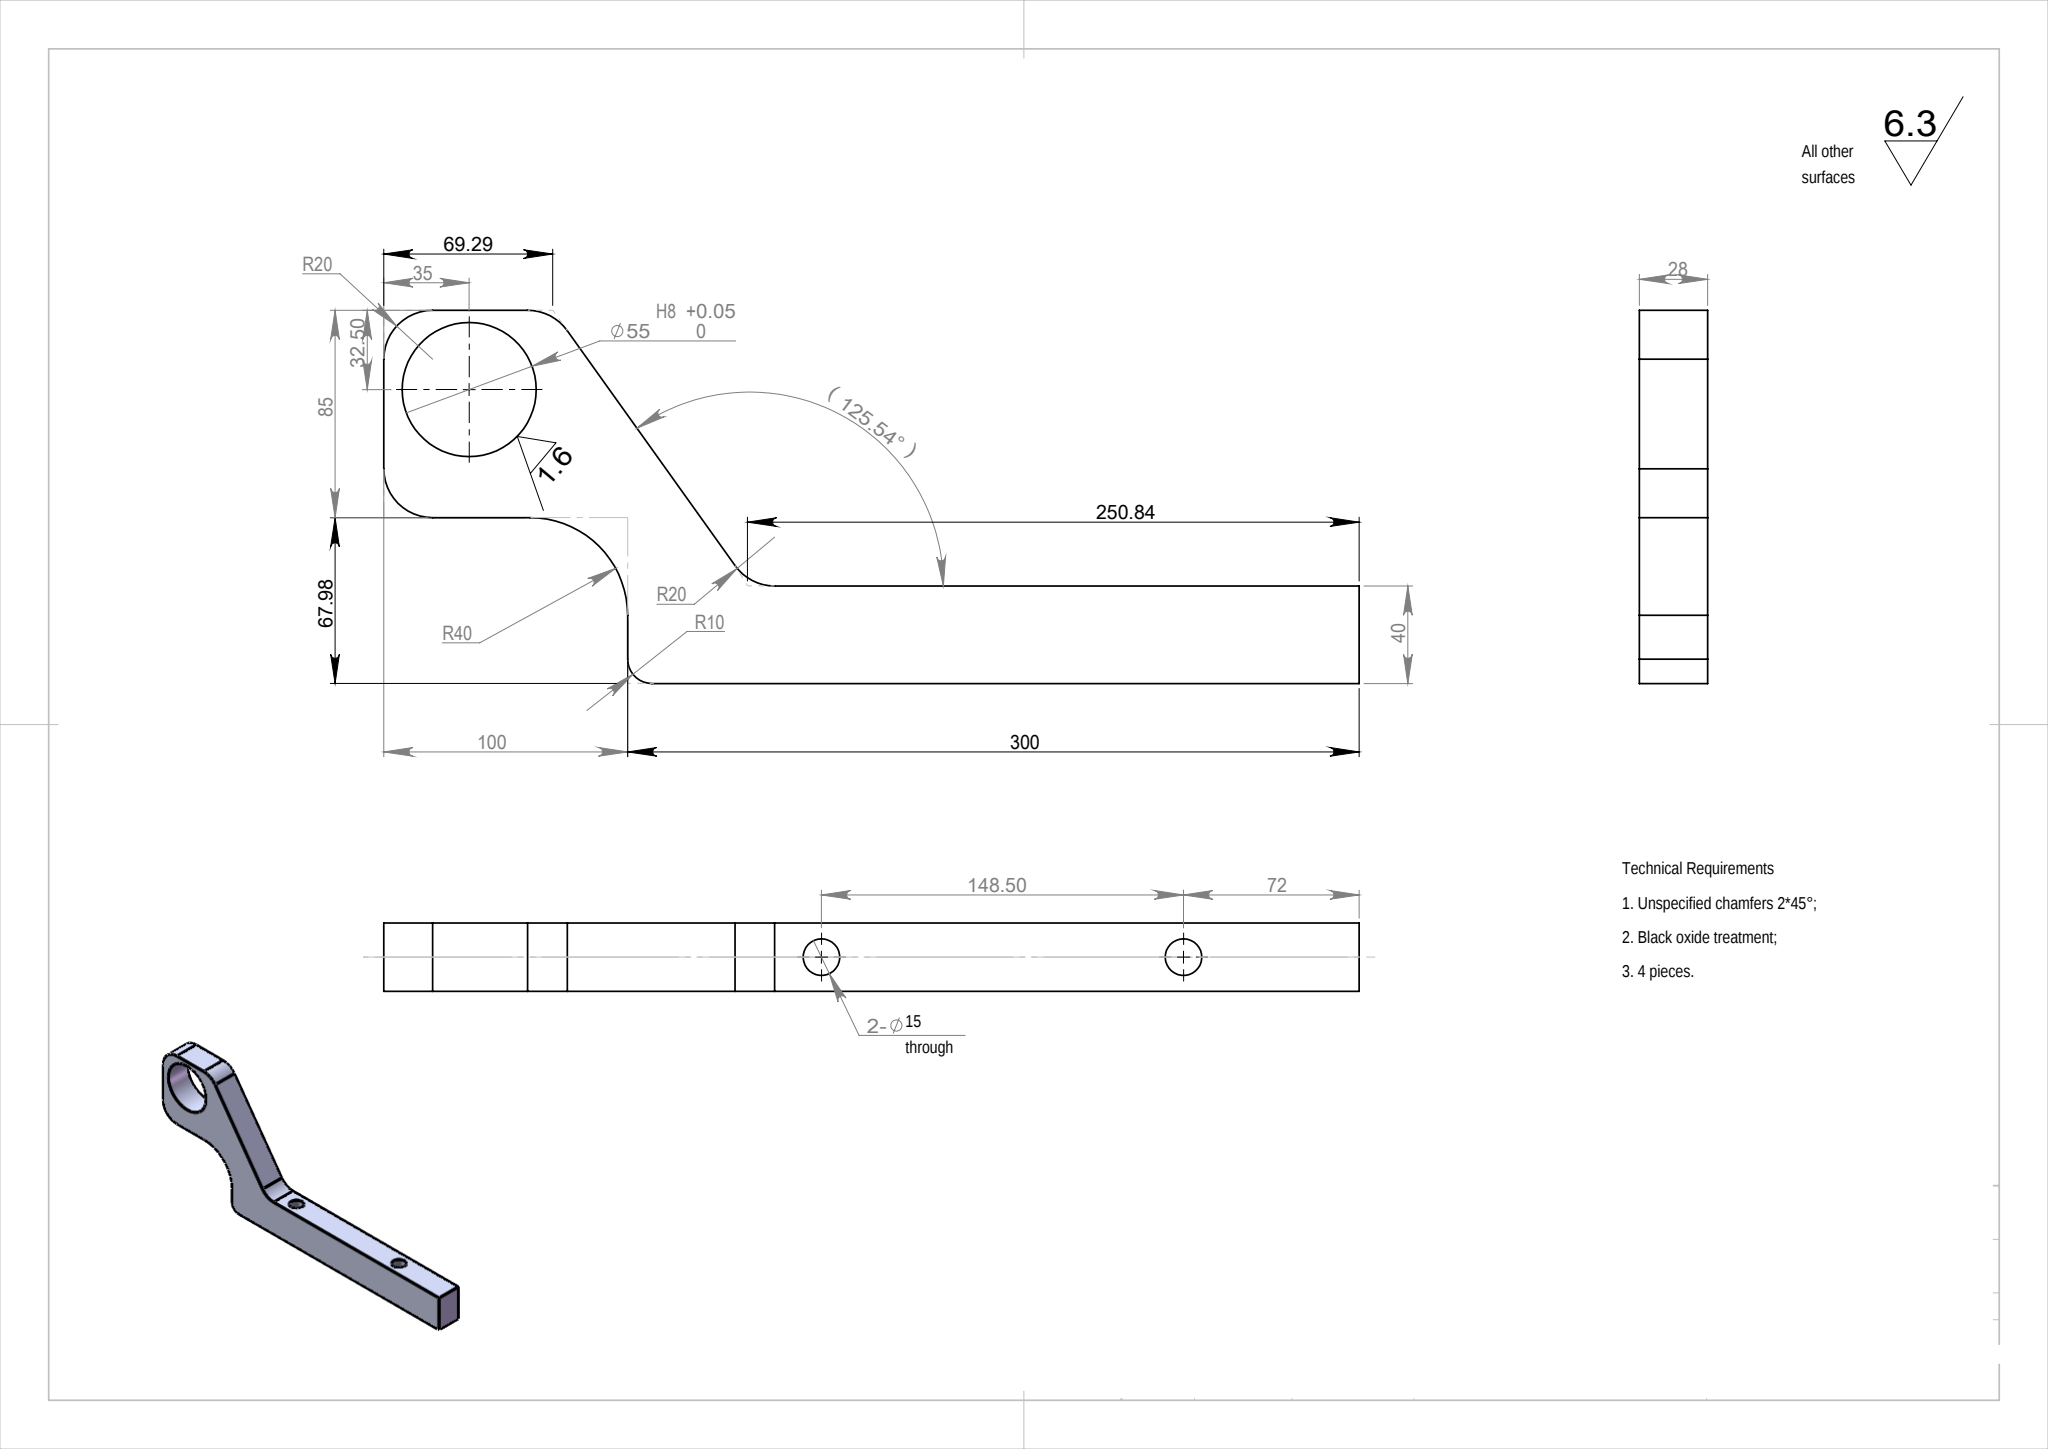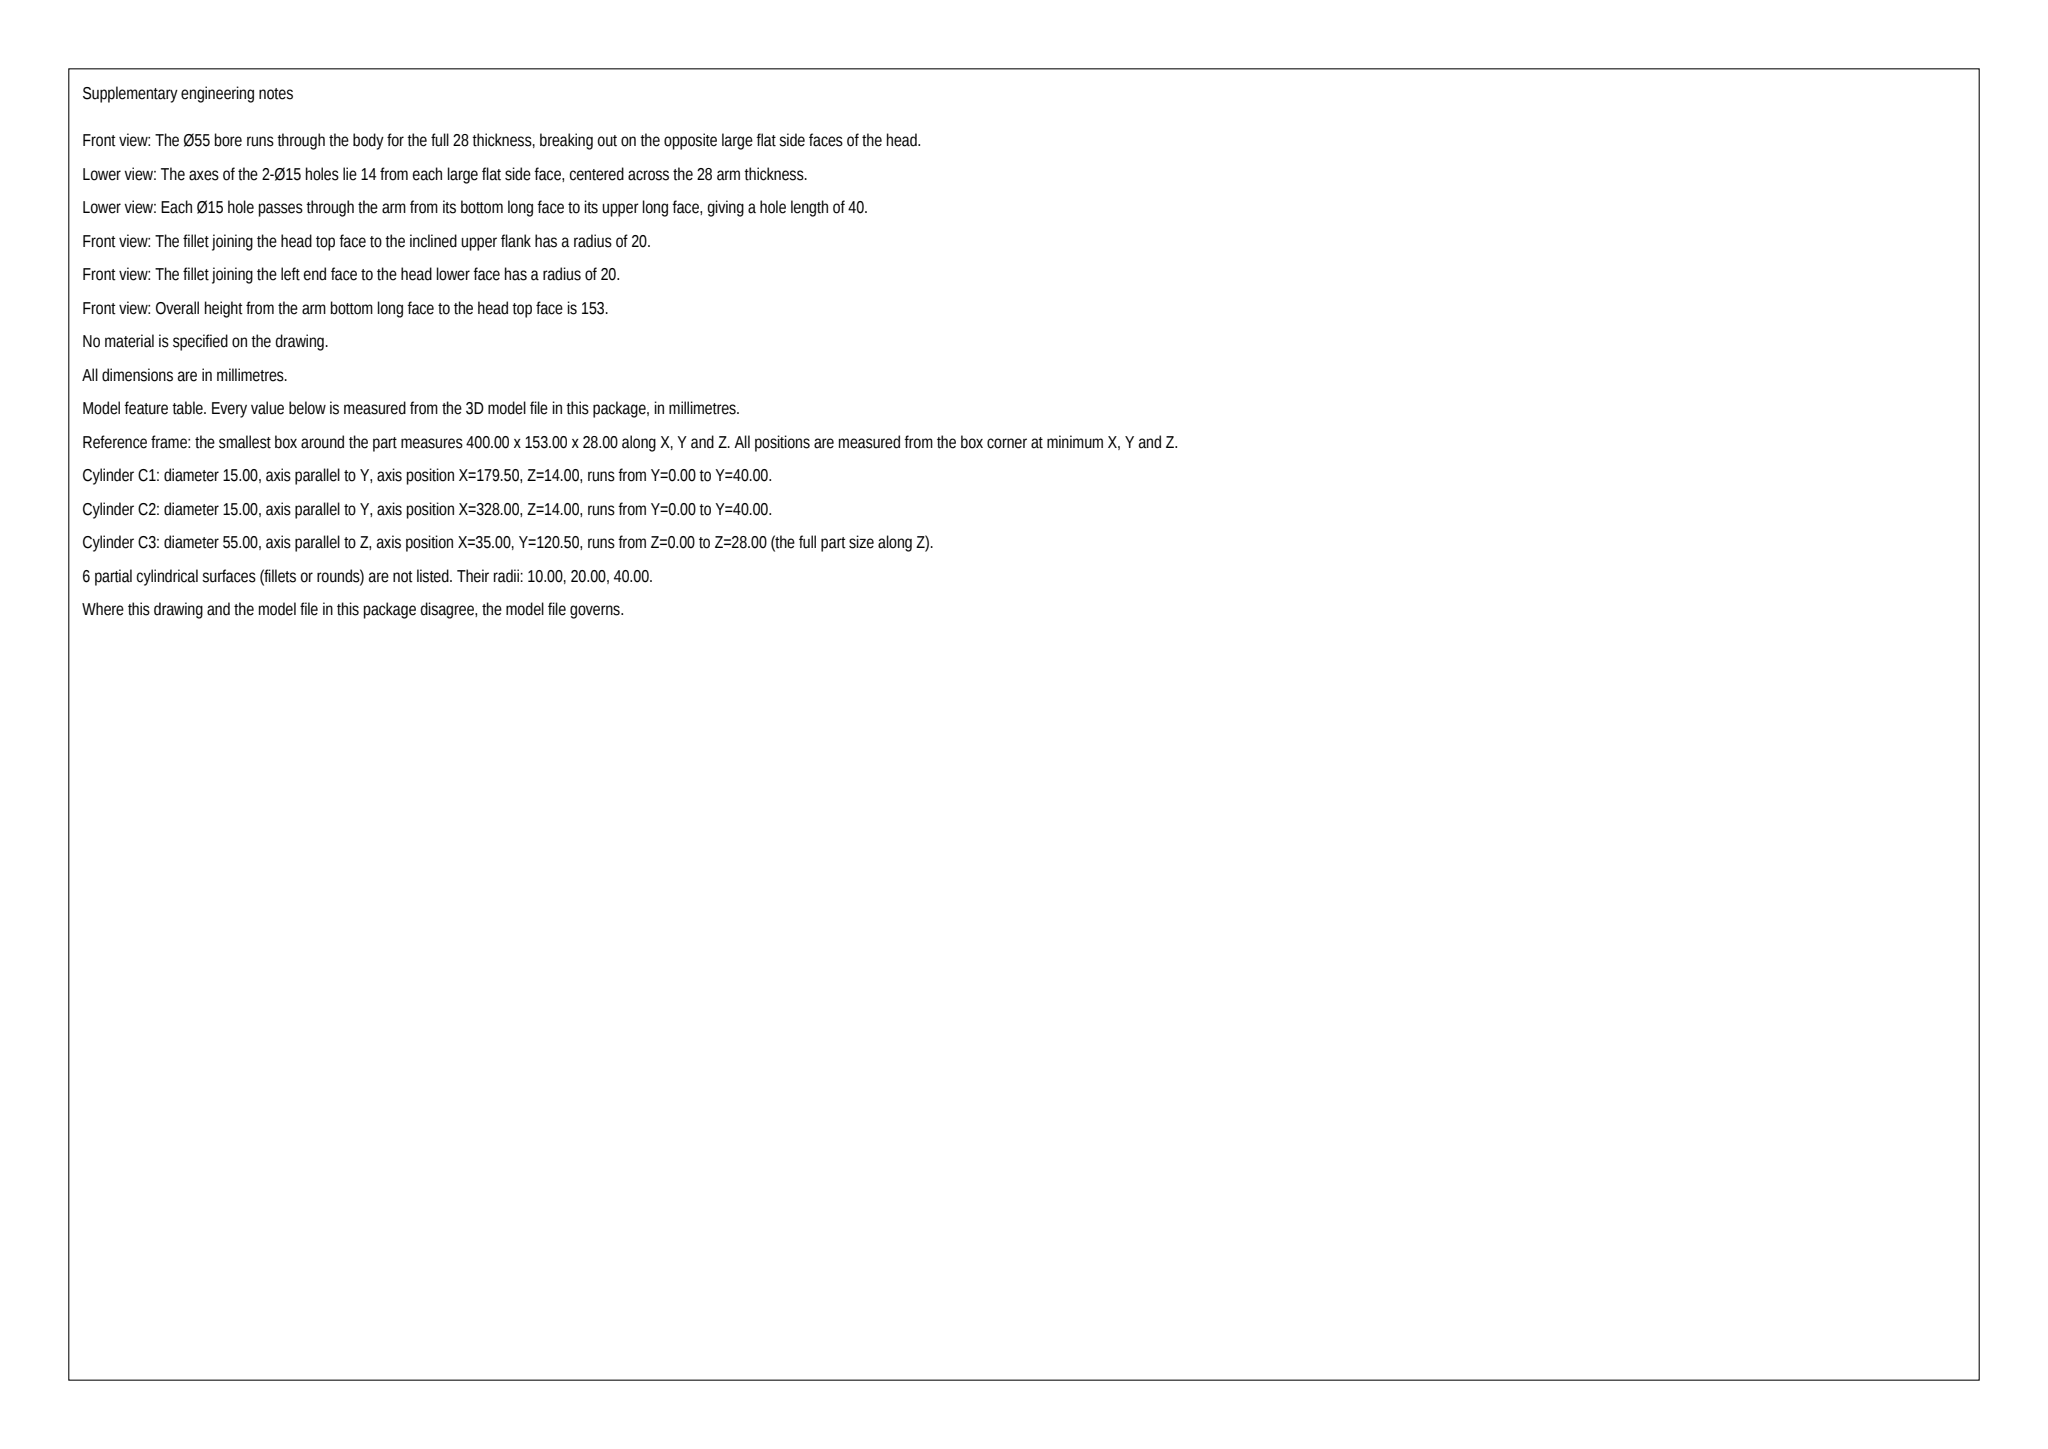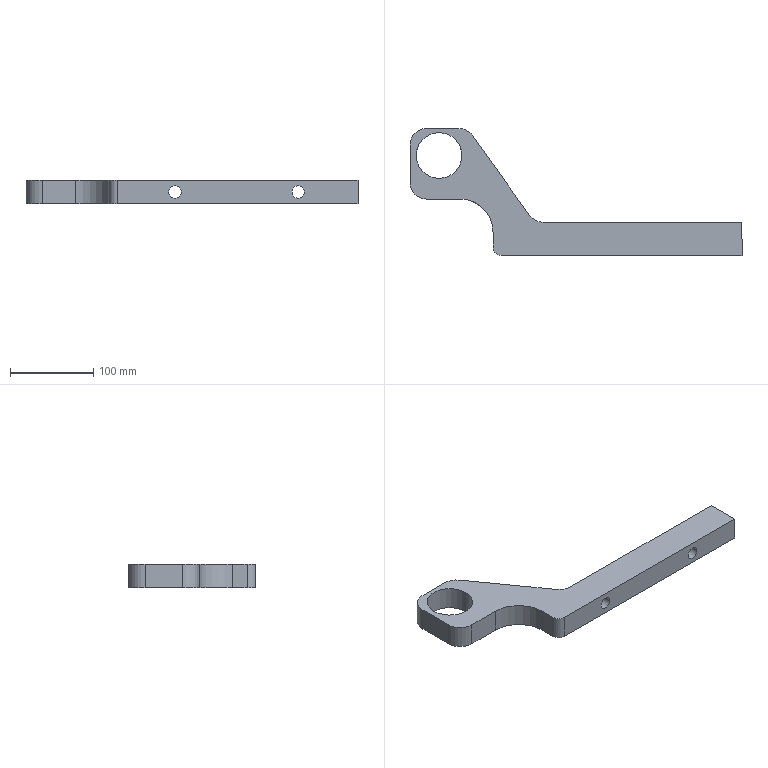Part | SolidWorks | mm | 1 solid | 22 faces | box 400 x 153 x 28 mm | volume 528056 mm3 | cylinder 12 | plane 10 | commonest cylinder face diameters 15 x4 40 x4 55 x2 80 x1 20 x1
Drawing notes:
FRONT VIEW: R20 AT LH END FACE/HEAD UNDERSIDE, CTR 20 FROM LH, 88 UP | from the solid: cylinder dia 40, axis z, pos (x=20, y=88), len 28 -> R20 tangent to planes x=0 and y=68
FRONT VIEW: R20 AT TOP EDGE/INCL EDGE, CTR 58.99 FROM LH, 133 UP | from the solid: cylinder dia 40, axis z, pos (x=58.99, y=133), len 28 -> R20 tangent to plane y=153 and inclined face
build123d program:
from build123d import *

# Parameters (mm, degrees)
BOSS_EXTRUDE1_DEPTH = 14
SKETCH2_R           = 5.5
CUT_EXTRUDE1_DEPTH  = 285.558
SKETCH3_R           = 27.5
CUT_EXTRUDE2_DEPTH  = 285.558
FILLET1_R           = 40
CUT_EXTRUDE5_DEPTH  = 285.558
FILLET3_R           = 20
FILLET5_R           = 10
CUT_EXTRUDE6_DEPTH  = 285.558
FILLET6_R           = 20
SKETCH13_R          = 7.5
CUT_EXTRUDE7_DEPTH  = 294.437


with BuildPart() as part:
    # Sketch1 → Boss-Extrude1 (new, symmetric)
    with BuildSketch(Plane.XY):
        Polygon((-150, 133), (0, 133), (0, 0), (250, 0), (250, -40), (-50, -40), (-50, 28), (-150, 28), align=None)
    extrude(amount=BOSS_EXTRUDE1_DEPTH, both=True)

    # Sketch2 → Cut-Extrude1 (cut, through all)
    with BuildSketch(Plane.XY.offset(14)):
        with Locations((-115, 80.5)):
            Circle(SKETCH2_R)
    extrude(amount=-CUT_EXTRUDE1_DEPTH, mode=Mode.SUBTRACT)

    # Sketch3 → Cut-Extrude2 (cut, through all)
    with BuildSketch(Plane(origin=(0, 0, 14), x_dir=(-1, 0, 0), z_dir=(0, 0, -1))):
        with Locations((115, 80.5)):
            Circle(SKETCH3_R)
    extrude(amount=CUT_EXTRUDE2_DEPTH, mode=Mode.SUBTRACT)

    # Fillet1
    fillet1_edges = [part.edges().sort_by_distance(p)[0] for p in [
        (-50, 28, 0),
    ]]
    fillet(fillet1_edges, radius=FILLET1_R)

    # Sketch10 → Cut-Extrude5 (cut, through all)
    with BuildSketch(Plane.XY.offset(14)):
        Polygon((-95, 133), (0, 0), (0, 133), align=None)
    extrude(amount=-CUT_EXTRUDE5_DEPTH, mode=Mode.SUBTRACT)

    # Fillet3
    fillet3_edges = [part.edges().sort_by_distance(p)[0] for p in [
        (0, 0, 0),
    ]]
    fillet(fillet3_edges, radius=FILLET3_R)

    # Fillet5
    fillet5_edges = [part.edges().sort_by_distance(p)[0] for p in [
        (-50, -40, 0),
    ]]
    fillet(fillet5_edges, radius=FILLET5_R)

    # Sketch11 → Cut-Extrude6 (cut, through all)
    with BuildSketch(Plane.XY.offset(14)):
        Polygon((-150, 113), (-80.714, 113), (-95, 133), (-150, 133), align=None)
    extrude(amount=-CUT_EXTRUDE6_DEPTH, mode=Mode.SUBTRACT)

    # Fillet6
    fillet6_edges = [part.edges().sort_by_distance(p)[0] for p in [
        (-150, 28, 0),
        (-150, 113, 0),
        (-80.714, 113, 0),
    ]]
    fillet(fillet6_edges, radius=FILLET6_R)

    # Sketch13 → Cut-Extrude7 (cut, through all)
    with BuildSketch(Plane.XZ.offset(40)):
        with Locations((29.5, 0)):
            Circle(SKETCH13_R)
        with Locations((178, 0)):
            Circle(SKETCH13_R)
    extrude(amount=-CUT_EXTRUDE7_DEPTH, mode=Mode.SUBTRACT)


solid = part.part
STEP:
#1=CARTESIAN_POINT('',(22.,0.,0.));
#2=VERTEX_POINT('',#1);
#3=CARTESIAN_POINT('',(37.,0.,0.));
#4=VERTEX_POINT('',#3);
#5=CARTESIAN_POINT('',(29.5,0.,0.));
#6=DIRECTION('',(0.,-1.,0.));
#7=DIRECTION('',(0.,0.,-1.));
#8=AXIS2_PLACEMENT_3D('',#5,#6,#7);
#9=CIRCLE('',#8,7.5);
#10=EDGE_CURVE('',#2,#4,#9,.T.);
#11=ORIENTED_EDGE('',*,*,#10,.F.);
#12=CARTESIAN_POINT('',(22.,-40.,0.));
#13=VERTEX_POINT('',#12);
#14=CARTESIAN_POINT('',(22.,113.,0.));
#15=DIRECTION('',(0.,-1.,0.));
#16=VECTOR('',#15,1000.);
#17=LINE('',#14,#16);
#18=EDGE_CURVE('',#2,#13,#17,.T.);
#19=ORIENTED_EDGE('',*,*,#18,.T.);
#20=CARTESIAN_POINT('',(37.,-40.,0.));
#21=VERTEX_POINT('',#20);
#22=CARTESIAN_POINT('',(29.5,-40.,0.));
#23=DIRECTION('',(0.,-1.,0.));
#24=DIRECTION('',(1.,0.,0.));
#25=AXIS2_PLACEMENT_3D('',#22,#23,#24);
#26=CIRCLE('',#25,7.5);
#27=EDGE_CURVE('',#13,#21,#26,.T.);
#28=ORIENTED_EDGE('',*,*,#27,.T.);
#29=CARTESIAN_POINT('',(37.,113.,0.));
#30=DIRECTION('',(0.,-1.,0.));
#31=VECTOR('',#30,1000.);
#32=LINE('',#29,#31);
#33=EDGE_CURVE('',#4,#21,#32,.T.);
#34=ORIENTED_EDGE('',*,*,#33,.F.);
#35=EDGE_LOOP('',(#11,#19,#28,#34));
#36=FACE_OUTER_BOUND('',#35,.T.);
#37=CARTESIAN_POINT('',(29.5,113.,0.));
#38=DIRECTION('',(0.,-1.,0.));
#39=DIRECTION('',(1.,0.,0.));
#40=AXIS2_PLACEMENT_3D('',#37,#38,#39);
#41=CYLINDRICAL_SURFACE('',#40,7.5);
#42=ADVANCED_FACE('',(#36),#41,.F.);
#43=CARTESIAN_POINT('',(170.5,0.,0.));
#44=VERTEX_POINT('',#43);
#45=CARTESIAN_POINT('',(185.5,0.,0.));
#46=VERTEX_POINT('',#45);
#47=CARTESIAN_POINT('',(178.,0.,0.));
#48=DIRECTION('',(0.,-1.,0.));
#49=DIRECTION('',(0.,0.,-1.));
#50=AXIS2_PLACEMENT_3D('',#47,#48,#49);
#51=CIRCLE('',#50,7.5);
#52=EDGE_CURVE('',#44,#46,#51,.T.);
#53=ORIENTED_EDGE('',*,*,#52,.F.);
#54=CARTESIAN_POINT('',(170.5,-40.,0.));
#55=VERTEX_POINT('',#54);
#56=CARTESIAN_POINT('',(170.5,113.,0.));
#57=DIRECTION('',(0.,-1.,0.));
#58=VECTOR('',#57,1000.);
#59=LINE('',#56,#58);
#60=EDGE_CURVE('',#44,#55,#59,.T.);
#61=ORIENTED_EDGE('',*,*,#60,.T.);
#62=CARTESIAN_POINT('',(185.5,-40.,0.));
#63=VERTEX_POINT('',#62);
#64=CARTESIAN_POINT('',(178.,-40.,0.));
#65=DIRECTION('',(0.,-1.,0.));
#66=DIRECTION('',(1.,0.,0.));
#67=AXIS2_PLACEMENT_3D('',#64,#65,#66);
#68=CIRCLE('',#67,7.5);
#69=EDGE_CURVE('',#55,#63,#68,.T.);
#70=ORIENTED_EDGE('',*,*,#69,.T.);
#71=CARTESIAN_POINT('',(185.5,113.,0.));
#72=DIRECTION('',(0.,-1.,0.));
#73=VECTOR('',#72,1000.);
#74=LINE('',#71,#73);
#75=EDGE_CURVE('',#46,#63,#74,.T.);
#76=ORIENTED_EDGE('',*,*,#75,.F.);
#77=EDGE_LOOP('',(#53,#61,#70,#76));
#78=FACE_OUTER_BOUND('',#77,.T.);
#79=CARTESIAN_POINT('',(178.,113.,0.));
#80=DIRECTION('',(0.,-1.,0.));
#81=DIRECTION('',(1.,0.,0.));
#82=AXIS2_PLACEMENT_3D('',#79,#80,#81);
#83=CYLINDRICAL_SURFACE('',#82,7.5);
#84=ADVANCED_FACE('',(#78),#83,.F.);
#85=CARTESIAN_POINT('',(-87.5,80.5,-14.));
#86=VERTEX_POINT('',#85);
#87=CARTESIAN_POINT('',(-142.5,80.5,-14.));
#88=VERTEX_POINT('',#87);
#89=CARTESIAN_POINT('',(-115.,80.5,-14.));
#90=DIRECTION('',(0.,0.,-1.));
#91=DIRECTION('',(-1.,0.,0.));
#92=AXIS2_PLACEMENT_3D('',#89,#90,#91);
#93=CIRCLE('',#92,27.5);
#94=EDGE_CURVE('',#86,#88,#93,.T.);
#95=ORIENTED_EDGE('',*,*,#94,.T.);
#96=CARTESIAN_POINT('',(-142.5,80.5,14.));
#97=VERTEX_POINT('',#96);
#98=CARTESIAN_POINT('',(-142.5,80.5,-14.));
#99=DIRECTION('',(0.,0.,1.));
#100=VECTOR('',#99,1000.);
#101=LINE('',#98,#100);
#102=EDGE_CURVE('',#88,#97,#101,.T.);
#103=ORIENTED_EDGE('',*,*,#102,.T.);
#104=CARTESIAN_POINT('',(-87.5,80.5,14.));
#105=VERTEX_POINT('',#104);
#106=CARTESIAN_POINT('',(-115.,80.5,14.));
#107=DIRECTION('',(0.,0.,-1.));
#108=DIRECTION('',(-1.,0.,0.));
#109=AXIS2_PLACEMENT_3D('',#106,#107,#108);
#110=CIRCLE('',#109,27.5);
#111=EDGE_CURVE('',#105,#97,#110,.T.);
#112=ORIENTED_EDGE('',*,*,#111,.F.);
#113=CARTESIAN_POINT('',(-87.5,80.5,-14.));
#114=DIRECTION('',(0.,0.,1.));
#115=VECTOR('',#114,1000.);
#116=LINE('',#113,#115);
#117=EDGE_CURVE('',#86,#105,#116,.T.);
#118=ORIENTED_EDGE('',*,*,#117,.F.);
#119=EDGE_LOOP('',(#95,#103,#112,#118));
#120=FACE_OUTER_BOUND('',#119,.T.);
#121=CARTESIAN_POINT('',(-115.,80.5,-14.));
#122=DIRECTION('',(0.,0.,1.));
#123=DIRECTION('',(1.,0.,0.));
#124=AXIS2_PLACEMENT_3D('',#121,#122,#123);
#125=CYLINDRICAL_SURFACE('',#124,27.5);
#126=ADVANCED_FACE('',(#120),#125,.F.);
#127=CARTESIAN_POINT('',(-150.,93.,14.));
#128=VERTEX_POINT('',#127);
#129=CARTESIAN_POINT('',(-150.,48.,14.));
#130=VERTEX_POINT('',#129);
#131=CARTESIAN_POINT('',(-150.,28.,14.));
#132=DIRECTION('',(-0.,-1.,0.));
#133=VECTOR('',#132,1000.);
#134=LINE('',#131,#133);
#135=EDGE_CURVE('',#128,#130,#134,.T.);
#136=ORIENTED_EDGE('',*,*,#135,.F.);
#137=CARTESIAN_POINT('',(-150.,93.,-14.));
#138=VERTEX_POINT('',#137);
#139=CARTESIAN_POINT('',(-150.,93.,14.));
#140=DIRECTION('',(0.,0.,-1.));
#141=VECTOR('',#140,1000.);
#142=LINE('',#139,#141);
#143=EDGE_CURVE('',#128,#138,#142,.T.);
#144=ORIENTED_EDGE('',*,*,#143,.T.);
#145=CARTESIAN_POINT('',(-150.,48.,-14.));
#146=VERTEX_POINT('',#145);
#147=CARTESIAN_POINT('',(-150.,28.,-14.));
#148=DIRECTION('',(-0.,-1.,0.));
#149=VECTOR('',#148,1000.);
#150=LINE('',#147,#149);
#151=EDGE_CURVE('',#138,#146,#150,.T.);
#152=ORIENTED_EDGE('',*,*,#151,.T.);
#153=CARTESIAN_POINT('',(-150.,48.,14.));
#154=DIRECTION('',(0.,0.,1.));
#155=VECTOR('',#154,1000.);
#156=LINE('',#153,#155);
#157=EDGE_CURVE('',#146,#130,#156,.T.);
#158=ORIENTED_EDGE('',*,*,#157,.T.);
#159=EDGE_LOOP('',(#136,#144,#152,#158));
#160=FACE_OUTER_BOUND('',#159,.T.);
#161=CARTESIAN_POINT('',(-150.,28.,14.));
#162=DIRECTION('',(1.,-0.,0.));
#163=DIRECTION('',(0.,1.,0.));
#164=AXIS2_PLACEMENT_3D('',#161,#162,#163);
#165=PLANE('',#164);
#166=ADVANCED_FACE('',(#160),#165,.F.);
#167=CARTESIAN_POINT('',(-130.,28.,14.));
#168=VERTEX_POINT('',#167);
#169=CARTESIAN_POINT('',(-90.,28.,14.));
#170=VERTEX_POINT('',#169);
#171=CARTESIAN_POINT('',(-50.,28.,14.));
#172=DIRECTION('',(1.,0.,0.));
#173=VECTOR('',#172,1000.);
#174=LINE('',#171,#173);
#175=EDGE_CURVE('',#168,#170,#174,.T.);
#176=ORIENTED_EDGE('',*,*,#175,.F.);
#177=CARTESIAN_POINT('',(-130.,28.,-14.));
#178=VERTEX_POINT('',#177);
#179=CARTESIAN_POINT('',(-130.,28.,14.));
#180=DIRECTION('',(0.,0.,-1.));
#181=VECTOR('',#180,1000.);
#182=LINE('',#179,#181);
#183=EDGE_CURVE('',#168,#178,#182,.T.);
#184=ORIENTED_EDGE('',*,*,#183,.T.);
#185=CARTESIAN_POINT('',(-90.,28.,-14.));
#186=VERTEX_POINT('',#185);
#187=CARTESIAN_POINT('',(-50.,28.,-14.));
#188=DIRECTION('',(1.,0.,0.));
#189=VECTOR('',#188,1000.);
#190=LINE('',#187,#189);
#191=EDGE_CURVE('',#178,#186,#190,.T.);
#192=ORIENTED_EDGE('',*,*,#191,.T.);
#193=CARTESIAN_POINT('',(-90.,28.,14.));
#194=DIRECTION('',(0.,0.,1.));
#195=VECTOR('',#194,1000.);
#196=LINE('',#193,#195);
#197=EDGE_CURVE('',#186,#170,#196,.T.);
#198=ORIENTED_EDGE('',*,*,#197,.T.);
#199=EDGE_LOOP('',(#176,#184,#192,#198));
#200=FACE_OUTER_BOUND('',#199,.T.);
#201=CARTESIAN_POINT('',(-50.,28.,14.));
#202=DIRECTION('',(-0.,1.,0.));
#203=DIRECTION('',(-1.,-0.,0.));
#204=AXIS2_PLACEMENT_3D('',#201,#202,#203);
#205=PLANE('',#204);
#206=ADVANCED_FACE('',(#200),#205,.F.);
#207=CARTESIAN_POINT('',(-50.,-12.,-14.));
#208=VERTEX_POINT('',#207);
#209=CARTESIAN_POINT('',(-50.,-30.,-14.));
#210=VERTEX_POINT('',#209);
#211=CARTESIAN_POINT('',(-50.,-40.,-14.));
#212=DIRECTION('',(0.,-1.,0.));
#213=VECTOR('',#212,1000.);
#214=LINE('',#211,#213);
#215=EDGE_CURVE('',#208,#210,#214,.T.);
#216=ORIENTED_EDGE('',*,*,#215,.T.);
#217=CARTESIAN_POINT('',(-50.,-30.,14.));
#218=VERTEX_POINT('',#217);
#219=CARTESIAN_POINT('',(-50.,-30.,14.));
#220=DIRECTION('',(0.,0.,1.));
#221=VECTOR('',#220,1000.);
#222=LINE('',#219,#221);
#223=EDGE_CURVE('',#210,#218,#222,.T.);
#224=ORIENTED_EDGE('',*,*,#223,.T.);
#225=CARTESIAN_POINT('',(-50.,-12.,14.));
#226=VERTEX_POINT('',#225);
#227=CARTESIAN_POINT('',(-50.,-40.,14.));
#228=DIRECTION('',(0.,-1.,0.));
#229=VECTOR('',#228,1000.);
#230=LINE('',#227,#229);
#231=EDGE_CURVE('',#226,#218,#230,.T.);
#232=ORIENTED_EDGE('',*,*,#231,.F.);
#233=CARTESIAN_POINT('',(-50.,-12.,-14.));
#234=DIRECTION('',(0.,0.,-1.));
#235=VECTOR('',#234,1000.);
#236=LINE('',#233,#235);
#237=EDGE_CURVE('',#226,#208,#236,.T.);
#238=ORIENTED_EDGE('',*,*,#237,.T.);
#239=EDGE_LOOP('',(#216,#224,#232,#238));
#240=FACE_OUTER_BOUND('',#239,.T.);
#241=CARTESIAN_POINT('',(-50.,-40.,14.));
#242=DIRECTION('',(1.,0.,0.));
#243=DIRECTION('',(-0.,1.,0.));
#244=AXIS2_PLACEMENT_3D('',#241,#242,#243);
#245=PLANE('',#244);
#246=ADVANCED_FACE('',(#240),#245,.F.);
#247=CARTESIAN_POINT('',(29.5,-40.,0.));
#248=DIRECTION('',(0.,-1.,0.));
#249=DIRECTION('',(1.,0.,0.));
#250=AXIS2_PLACEMENT_3D('',#247,#248,#249);
#251=CIRCLE('',#250,7.5);
#252=EDGE_CURVE('',#21,#13,#251,.T.);
#253=ORIENTED_EDGE('',*,*,#252,.F.);
#254=ORIENTED_EDGE('',*,*,#27,.F.);
#255=EDGE_LOOP('',(#253,#254));
#256=FACE_BOUND('',#255,.T.);
#257=CARTESIAN_POINT('',(178.,-40.,0.));
#258=DIRECTION('',(0.,-1.,0.));
#259=DIRECTION('',(1.,0.,0.));
#260=AXIS2_PLACEMENT_3D('',#257,#258,#259);
#261=CIRCLE('',#260,7.5);
#262=EDGE_CURVE('',#63,#55,#261,.T.);
#263=ORIENTED_EDGE('',*,*,#262,.F.);
#264=ORIENTED_EDGE('',*,*,#69,.F.);
#265=EDGE_LOOP('',(#263,#264));
#266=FACE_BOUND('',#265,.T.);
#267=CARTESIAN_POINT('',(-40.,-40.,14.));
#268=VERTEX_POINT('',#267);
#269=CARTESIAN_POINT('',(250.,-40.,14.));
#270=VERTEX_POINT('',#269);
#271=CARTESIAN_POINT('',(250.,-40.,14.));
#272=DIRECTION('',(1.,0.,0.));
#273=VECTOR('',#272,1000.);
#274=LINE('',#271,#273);
#275=EDGE_CURVE('',#268,#270,#274,.T.);
#276=ORIENTED_EDGE('',*,*,#275,.F.);
#277=CARTESIAN_POINT('',(-40.,-40.,-14.));
#278=VERTEX_POINT('',#277);
#279=CARTESIAN_POINT('',(-40.,-40.,14.));
#280=DIRECTION('',(0.,0.,-1.));
#281=VECTOR('',#280,1000.);
#282=LINE('',#279,#281);
#283=EDGE_CURVE('',#268,#278,#282,.T.);
#284=ORIENTED_EDGE('',*,*,#283,.T.);
#285=CARTESIAN_POINT('',(250.,-40.,-14.));
#286=VERTEX_POINT('',#285);
#287=CARTESIAN_POINT('',(250.,-40.,-14.));
#288=DIRECTION('',(1.,0.,0.));
#289=VECTOR('',#288,1000.);
#290=LINE('',#287,#289);
#291=EDGE_CURVE('',#278,#286,#290,.T.);
#292=ORIENTED_EDGE('',*,*,#291,.T.);
#293=CARTESIAN_POINT('',(250.,-40.,14.));
#294=DIRECTION('',(0.,0.,-1.));
#295=VECTOR('',#294,1000.);
#296=LINE('',#293,#295);
#297=EDGE_CURVE('',#270,#286,#296,.T.);
#298=ORIENTED_EDGE('',*,*,#297,.F.);
#299=EDGE_LOOP('',(#276,#284,#292,#298));
#300=FACE_OUTER_BOUND('',#299,.T.);
#301=CARTESIAN_POINT('',(250.,-40.,14.));
#302=DIRECTION('',(-0.,1.,0.));
#303=DIRECTION('',(-1.,-0.,0.));
#304=AXIS2_PLACEMENT_3D('',#301,#302,#303);
#305=PLANE('',#304);
#306=ADVANCED_FACE('',(#256,#266,#300),#305,.F.);
#307=CARTESIAN_POINT('',(250.,0.,-14.));
#308=VERTEX_POINT('',#307);
#309=CARTESIAN_POINT('',(250.,0.,-14.));
#310=DIRECTION('',(-0.,1.,0.));
#311=VECTOR('',#310,1000.);
#312=LINE('',#309,#311);
#313=EDGE_CURVE('',#286,#308,#312,.T.);
#314=ORIENTED_EDGE('',*,*,#313,.T.);
#315=CARTESIAN_POINT('',(250.,0.,14.));
#316=VERTEX_POINT('',#315);
#317=CARTESIAN_POINT('',(250.,0.,14.));
#318=DIRECTION('',(0.,0.,-1.));
#319=VECTOR('',#318,1000.);
#320=LINE('',#317,#319);
#321=EDGE_CURVE('',#316,#308,#320,.T.);
#322=ORIENTED_EDGE('',*,*,#321,.F.);
#323=CARTESIAN_POINT('',(250.,0.,14.));
#324=DIRECTION('',(-0.,1.,0.));
#325=VECTOR('',#324,1000.);
#326=LINE('',#323,#325);
#327=EDGE_CURVE('',#270,#316,#326,.T.);
#328=ORIENTED_EDGE('',*,*,#327,.F.);
#329=ORIENTED_EDGE('',*,*,#297,.T.);
#330=EDGE_LOOP('',(#314,#322,#328,#329));
#331=FACE_OUTER_BOUND('',#330,.T.);
#332=CARTESIAN_POINT('',(250.,0.,14.));
#333=DIRECTION('',(-1.,-0.,0.));
#334=DIRECTION('',(0.,-1.,0.));
#335=AXIS2_PLACEMENT_3D('',#332,#333,#334);
#336=PLANE('',#335);
#337=ADVANCED_FACE('',(#331),#336,.F.);
#338=CARTESIAN_POINT('',(29.5,0.,0.));
#339=DIRECTION('',(0.,-1.,0.));
#340=DIRECTION('',(0.,0.,-1.));
#341=AXIS2_PLACEMENT_3D('',#338,#339,#340);
#342=CIRCLE('',#341,7.5);
#343=EDGE_CURVE('',#4,#2,#342,.T.);
#344=ORIENTED_EDGE('',*,*,#343,.T.);
#345=ORIENTED_EDGE('',*,*,#10,.T.);
#346=EDGE_LOOP('',(#344,#345));
#347=FACE_BOUND('',#346,.T.);
#348=CARTESIAN_POINT('',(178.,0.,0.));
#349=DIRECTION('',(0.,-1.,0.));
#350=DIRECTION('',(0.,0.,-1.));
#351=AXIS2_PLACEMENT_3D('',#348,#349,#350);
#352=CIRCLE('',#351,7.5);
#353=EDGE_CURVE('',#46,#44,#352,.T.);
#354=ORIENTED_EDGE('',*,*,#353,.T.);
#355=ORIENTED_EDGE('',*,*,#52,.T.);
#356=EDGE_LOOP('',(#354,#355));
#357=FACE_BOUND('',#356,.T.);
#358=CARTESIAN_POINT('',(10.292,0.,-14.));
#359=VERTEX_POINT('',#358);
#360=CARTESIAN_POINT('',(0.,0.,-14.));
#361=DIRECTION('',(-1.,0.,0.));
#362=VECTOR('',#361,1000.);
#363=LINE('',#360,#362);
#364=EDGE_CURVE('',#308,#359,#363,.T.);
#365=ORIENTED_EDGE('',*,*,#364,.T.);
#366=CARTESIAN_POINT('',(10.292,0.,14.));
#367=VERTEX_POINT('',#366);
#368=CARTESIAN_POINT('',(10.292,0.,14.));
#369=DIRECTION('',(0.,0.,1.));
#370=VECTOR('',#369,1000.);
#371=LINE('',#368,#370);
#372=EDGE_CURVE('',#359,#367,#371,.T.);
#373=ORIENTED_EDGE('',*,*,#372,.T.);
#374=CARTESIAN_POINT('',(0.,0.,14.));
#375=DIRECTION('',(-1.,0.,0.));
#376=VECTOR('',#375,1000.);
#377=LINE('',#374,#376);
#378=EDGE_CURVE('',#316,#367,#377,.T.);
#379=ORIENTED_EDGE('',*,*,#378,.F.);
#380=ORIENTED_EDGE('',*,*,#321,.T.);
#381=EDGE_LOOP('',(#365,#373,#379,#380));
#382=FACE_OUTER_BOUND('',#381,.T.);
#383=CARTESIAN_POINT('',(0.,0.,14.));
#384=DIRECTION('',(0.,-1.,0.));
#385=DIRECTION('',(0.,0.,-1.));
#386=AXIS2_PLACEMENT_3D('',#383,#384,#385);
#387=PLANE('',#386);
#388=ADVANCED_FACE('',(#347,#357,#382),#387,.F.);
#389=ORIENTED_EDGE('',*,*,#111,.T.);
#390=CARTESIAN_POINT('',(-115.,80.5,14.));
#391=DIRECTION('',(0.,0.,-1.));
#392=DIRECTION('',(-1.,0.,0.));
#393=AXIS2_PLACEMENT_3D('',#390,#391,#392);
#394=CIRCLE('',#393,27.5);
#395=EDGE_CURVE('',#97,#105,#394,.T.);
#396=ORIENTED_EDGE('',*,*,#395,.T.);
#397=EDGE_LOOP('',(#389,#396));
#398=FACE_BOUND('',#397,.T.);
#399=CARTESIAN_POINT('',(-130.,113.,14.));
#400=VERTEX_POINT('',#399);
#401=CARTESIAN_POINT('',(-91.007,113.,14.));
#402=VERTEX_POINT('',#401);
#403=CARTESIAN_POINT('',(-150.,113.,14.));
#404=DIRECTION('',(1.,0.,0.));
#405=VECTOR('',#404,1000.);
#406=LINE('',#403,#405);
#407=EDGE_CURVE('',#400,#402,#406,.T.);
#408=ORIENTED_EDGE('',*,*,#407,.F.);
#409=CARTESIAN_POINT('',(-130.,93.,14.));
#410=DIRECTION('',(0.,0.,1.));
#411=DIRECTION('',(-1.,0.,0.));
#412=AXIS2_PLACEMENT_3D('',#409,#410,#411);
#413=CIRCLE('',#412,20.);
#414=EDGE_CURVE('',#400,#128,#413,.T.);
#415=ORIENTED_EDGE('',*,*,#414,.T.);
#416=ORIENTED_EDGE('',*,*,#135,.T.);
#417=CARTESIAN_POINT('',(-130.,48.,14.));
#418=DIRECTION('',(0.,0.,1.));
#419=DIRECTION('',(-1.,0.,0.));
#420=AXIS2_PLACEMENT_3D('',#417,#418,#419);
#421=CIRCLE('',#420,20.);
#422=EDGE_CURVE('',#130,#168,#421,.T.);
#423=ORIENTED_EDGE('',*,*,#422,.T.);
#424=ORIENTED_EDGE('',*,*,#175,.T.);
#425=CARTESIAN_POINT('',(-90.,-12.,14.));
#426=DIRECTION('',(0.,0.,-1.));
#427=DIRECTION('',(-1.,0.,0.));
#428=AXIS2_PLACEMENT_3D('',#425,#426,#427);
#429=CIRCLE('',#428,40.);
#430=EDGE_CURVE('',#170,#226,#429,.T.);
#431=ORIENTED_EDGE('',*,*,#430,.T.);
#432=ORIENTED_EDGE('',*,*,#231,.T.);
#433=CARTESIAN_POINT('',(-40.,-30.,14.));
#434=DIRECTION('',(0.,0.,1.));
#435=DIRECTION('',(-1.,0.,0.));
#436=AXIS2_PLACEMENT_3D('',#433,#434,#435);
#437=CIRCLE('',#436,10.);
#438=EDGE_CURVE('',#218,#268,#437,.T.);
#439=ORIENTED_EDGE('',*,*,#438,.T.);
#440=ORIENTED_EDGE('',*,*,#275,.T.);
#441=ORIENTED_EDGE('',*,*,#327,.T.);
#442=ORIENTED_EDGE('',*,*,#378,.T.);
#443=CARTESIAN_POINT('',(-5.982,8.375,14.));
#444=VERTEX_POINT('',#443);
#445=CARTESIAN_POINT('',(10.292,20.,14.));
#446=DIRECTION('',(0.,0.,-1.));
#447=DIRECTION('',(-1.,0.,0.));
#448=AXIS2_PLACEMENT_3D('',#445,#446,#447);
#449=CIRCLE('',#448,20.);
#450=EDGE_CURVE('',#367,#444,#449,.T.);
#451=ORIENTED_EDGE('',*,*,#450,.T.);
#452=CARTESIAN_POINT('',(-74.732,104.625,14.));
#453=VERTEX_POINT('',#452);
#454=CARTESIAN_POINT('',(-95.,133.,14.));
#455=DIRECTION('',(0.5812,-0.8137,0.));
#456=VECTOR('',#455,1000.);
#457=LINE('',#454,#456);
#458=EDGE_CURVE('',#453,#444,#457,.T.);
#459=ORIENTED_EDGE('',*,*,#458,.F.);
#460=CARTESIAN_POINT('',(-91.007,93.,14.));
#461=DIRECTION('',(0.,0.,1.));
#462=DIRECTION('',(-1.,0.,0.));
#463=AXIS2_PLACEMENT_3D('',#460,#461,#462);
#464=CIRCLE('',#463,20.);
#465=EDGE_CURVE('',#453,#402,#464,.T.);
#466=ORIENTED_EDGE('',*,*,#465,.T.);
#467=EDGE_LOOP('',(#408,#415,#416,#423,#424,#431,#432,#439,#440,#441,#442,#451,#459,#466));
#468=FACE_OUTER_BOUND('',#467,.T.);
#469=CARTESIAN_POINT('',(0.,0.,14.));
#470=DIRECTION('',(0.,0.,-1.));
#471=DIRECTION('',(-1.,0.,0.));
#472=AXIS2_PLACEMENT_3D('',#469,#470,#471);
#473=PLANE('',#472);
#474=ADVANCED_FACE('',(#398,#468),#473,.F.);
#475=ORIENTED_EDGE('',*,*,#151,.F.);
#476=CARTESIAN_POINT('',(-130.,113.,-14.));
#477=VERTEX_POINT('',#476);
#478=CARTESIAN_POINT('',(-130.,93.,-14.));
#479=DIRECTION('',(0.,0.,-1.));
#480=DIRECTION('',(-1.,0.,0.));
#481=AXIS2_PLACEMENT_3D('',#478,#479,#480);
#482=CIRCLE('',#481,20.);
#483=EDGE_CURVE('',#138,#477,#482,.T.);
#484=ORIENTED_EDGE('',*,*,#483,.T.);
#485=CARTESIAN_POINT('',(-91.007,113.,-14.));
#486=VERTEX_POINT('',#485);
#487=CARTESIAN_POINT('',(-150.,113.,-14.));
#488=DIRECTION('',(1.,0.,0.));
#489=VECTOR('',#488,1000.);
#490=LINE('',#487,#489);
#491=EDGE_CURVE('',#477,#486,#490,.T.);
#492=ORIENTED_EDGE('',*,*,#491,.T.);
#493=CARTESIAN_POINT('',(-74.732,104.625,-14.));
#494=VERTEX_POINT('',#493);
#495=CARTESIAN_POINT('',(-91.007,93.,-14.));
#496=DIRECTION('',(0.,0.,-1.));
#497=DIRECTION('',(-1.,0.,0.));
#498=AXIS2_PLACEMENT_3D('',#495,#496,#497);
#499=CIRCLE('',#498,20.);
#500=EDGE_CURVE('',#486,#494,#499,.T.);
#501=ORIENTED_EDGE('',*,*,#500,.T.);
#502=CARTESIAN_POINT('',(-5.982,8.375,-14.));
#503=VERTEX_POINT('',#502);
#504=CARTESIAN_POINT('',(-95.,133.,-14.));
#505=DIRECTION('',(0.5812,-0.8137,0.));
#506=VECTOR('',#505,1000.);
#507=LINE('',#504,#506);
#508=EDGE_CURVE('',#494,#503,#507,.T.);
#509=ORIENTED_EDGE('',*,*,#508,.T.);
#510=CARTESIAN_POINT('',(10.292,20.,-14.));
#511=DIRECTION('',(0.,0.,1.));
#512=DIRECTION('',(-1.,0.,0.));
#513=AXIS2_PLACEMENT_3D('',#510,#511,#512);
#514=CIRCLE('',#513,20.);
#515=EDGE_CURVE('',#503,#359,#514,.T.);
#516=ORIENTED_EDGE('',*,*,#515,.T.);
#517=ORIENTED_EDGE('',*,*,#364,.F.);
#518=ORIENTED_EDGE('',*,*,#313,.F.);
#519=ORIENTED_EDGE('',*,*,#291,.F.);
#520=CARTESIAN_POINT('',(-40.,-30.,-14.));
#521=DIRECTION('',(0.,0.,-1.));
#522=DIRECTION('',(-1.,0.,0.));
#523=AXIS2_PLACEMENT_3D('',#520,#521,#522);
#524=CIRCLE('',#523,10.);
#525=EDGE_CURVE('',#278,#210,#524,.T.);
#526=ORIENTED_EDGE('',*,*,#525,.T.);
#527=ORIENTED_EDGE('',*,*,#215,.F.);
#528=CARTESIAN_POINT('',(-90.,-12.,-14.));
#529=DIRECTION('',(0.,0.,1.));
#530=DIRECTION('',(-1.,0.,0.));
#531=AXIS2_PLACEMENT_3D('',#528,#529,#530);
#532=CIRCLE('',#531,40.);
#533=EDGE_CURVE('',#208,#186,#532,.T.);
#534=ORIENTED_EDGE('',*,*,#533,.T.);
#535=ORIENTED_EDGE('',*,*,#191,.F.);
#536=CARTESIAN_POINT('',(-130.,48.,-14.));
#537=DIRECTION('',(0.,0.,-1.));
#538=DIRECTION('',(-1.,0.,0.));
#539=AXIS2_PLACEMENT_3D('',#536,#537,#538);
#540=CIRCLE('',#539,20.);
#541=EDGE_CURVE('',#178,#146,#540,.T.);
#542=ORIENTED_EDGE('',*,*,#541,.T.);
#543=EDGE_LOOP('',(#475,#484,#492,#501,#509,#516,#517,#518,#519,#526,#527,#534,#535,#542));
#544=FACE_OUTER_BOUND('',#543,.T.);
#545=ORIENTED_EDGE('',*,*,#94,.F.);
#546=CARTESIAN_POINT('',(-115.,80.5,-14.));
#547=DIRECTION('',(0.,0.,-1.));
#548=DIRECTION('',(-1.,0.,0.));
#549=AXIS2_PLACEMENT_3D('',#546,#547,#548);
#550=CIRCLE('',#549,27.5);
#551=EDGE_CURVE('',#88,#86,#550,.T.);
#552=ORIENTED_EDGE('',*,*,#551,.F.);
#553=EDGE_LOOP('',(#545,#552));
#554=FACE_BOUND('',#553,.T.);
#555=CARTESIAN_POINT('',(0.,0.,-14.));
#556=DIRECTION('',(0.,0.,-1.));
#557=DIRECTION('',(-1.,0.,0.));
#558=AXIS2_PLACEMENT_3D('',#555,#556,#557);
#559=PLANE('',#558);
#560=ADVANCED_FACE('',(#544,#554),#559,.T.);
#561=ORIENTED_EDGE('',*,*,#102,.F.);
#562=ORIENTED_EDGE('',*,*,#551,.T.);
#563=ORIENTED_EDGE('',*,*,#117,.T.);
#564=ORIENTED_EDGE('',*,*,#395,.F.);
#565=EDGE_LOOP('',(#561,#562,#563,#564));
#566=FACE_OUTER_BOUND('',#565,.T.);
#567=CARTESIAN_POINT('',(-115.,80.5,-14.));
#568=DIRECTION('',(0.,0.,1.));
#569=DIRECTION('',(1.,0.,0.));
#570=AXIS2_PLACEMENT_3D('',#567,#568,#569);
#571=CYLINDRICAL_SURFACE('',#570,27.5);
#572=ADVANCED_FACE('',(#566),#571,.F.);
#573=ORIENTED_EDGE('',*,*,#430,.F.);
#574=ORIENTED_EDGE('',*,*,#197,.F.);
#575=ORIENTED_EDGE('',*,*,#533,.F.);
#576=ORIENTED_EDGE('',*,*,#237,.F.);
#577=EDGE_LOOP('',(#573,#574,#575,#576));
#578=FACE_OUTER_BOUND('',#577,.T.);
#579=CARTESIAN_POINT('',(-90.,-12.,14.));
#580=DIRECTION('',(0.,0.,1.));
#581=DIRECTION('',(1.,0.,0.));
#582=AXIS2_PLACEMENT_3D('',#579,#580,#581);
#583=CYLINDRICAL_SURFACE('',#582,40.);
#584=ADVANCED_FACE('',(#578),#583,.F.);
#585=ORIENTED_EDGE('',*,*,#508,.F.);
#586=CARTESIAN_POINT('',(-74.732,104.625,-14.));
#587=DIRECTION('',(0.,0.,1.));
#588=VECTOR('',#587,1000.);
#589=LINE('',#586,#588);
#590=EDGE_CURVE('',#494,#453,#589,.T.);
#591=ORIENTED_EDGE('',*,*,#590,.T.);
#592=ORIENTED_EDGE('',*,*,#458,.T.);
#593=CARTESIAN_POINT('',(-5.982,8.375,-14.));
#594=DIRECTION('',(0.,0.,-1.));
#595=VECTOR('',#594,1000.);
#596=LINE('',#593,#595);
#597=EDGE_CURVE('',#444,#503,#596,.T.);
#598=ORIENTED_EDGE('',*,*,#597,.T.);
#599=EDGE_LOOP('',(#585,#591,#592,#598));
#600=FACE_OUTER_BOUND('',#599,.T.);
#601=CARTESIAN_POINT('',(-95.,133.,-14.));
#602=DIRECTION('',(-0.8137,-0.5812,0.));
#603=DIRECTION('',(0.5812,-0.8137,0.));
#604=AXIS2_PLACEMENT_3D('',#601,#602,#603);
#605=PLANE('',#604);
#606=ADVANCED_FACE('',(#600),#605,.F.);
#607=ORIENTED_EDGE('',*,*,#450,.F.);
#608=ORIENTED_EDGE('',*,*,#372,.F.);
#609=ORIENTED_EDGE('',*,*,#515,.F.);
#610=ORIENTED_EDGE('',*,*,#597,.F.);
#611=EDGE_LOOP('',(#607,#608,#609,#610));
#612=FACE_OUTER_BOUND('',#611,.T.);
#613=CARTESIAN_POINT('',(10.292,20.,-14.));
#614=DIRECTION('',(0.,0.,1.));
#615=DIRECTION('',(1.,0.,0.));
#616=AXIS2_PLACEMENT_3D('',#613,#614,#615);
#617=CYLINDRICAL_SURFACE('',#616,20.);
#618=ADVANCED_FACE('',(#612),#617,.F.);
#619=ORIENTED_EDGE('',*,*,#438,.F.);
#620=ORIENTED_EDGE('',*,*,#223,.F.);
#621=ORIENTED_EDGE('',*,*,#525,.F.);
#622=ORIENTED_EDGE('',*,*,#283,.F.);
#623=EDGE_LOOP('',(#619,#620,#621,#622));
#624=FACE_OUTER_BOUND('',#623,.T.);
#625=CARTESIAN_POINT('',(-40.,-30.,14.));
#626=DIRECTION('',(0.,0.,-1.));
#627=DIRECTION('',(-1.,0.,0.));
#628=AXIS2_PLACEMENT_3D('',#625,#626,#627);
#629=CYLINDRICAL_SURFACE('',#628,10.);
#630=ADVANCED_FACE('',(#624),#629,.T.);
#631=ORIENTED_EDGE('',*,*,#491,.F.);
#632=CARTESIAN_POINT('',(-130.,113.,-14.));
#633=DIRECTION('',(0.,0.,1.));
#634=VECTOR('',#633,1000.);
#635=LINE('',#632,#634);
#636=EDGE_CURVE('',#477,#400,#635,.T.);
#637=ORIENTED_EDGE('',*,*,#636,.T.);
#638=ORIENTED_EDGE('',*,*,#407,.T.);
#639=CARTESIAN_POINT('',(-91.007,113.,-14.));
#640=DIRECTION('',(0.,0.,-1.));
#641=VECTOR('',#640,1000.);
#642=LINE('',#639,#641);
#643=EDGE_CURVE('',#402,#486,#642,.T.);
#644=ORIENTED_EDGE('',*,*,#643,.T.);
#645=EDGE_LOOP('',(#631,#637,#638,#644));
#646=FACE_OUTER_BOUND('',#645,.T.);
#647=CARTESIAN_POINT('',(-150.,113.,-14.));
#648=DIRECTION('',(0.,-1.,0.));
#649=DIRECTION('',(0.,0.,-1.));
#650=AXIS2_PLACEMENT_3D('',#647,#648,#649);
#651=PLANE('',#650);
#652=ADVANCED_FACE('',(#646),#651,.F.);
#653=ORIENTED_EDGE('',*,*,#483,.F.);
#654=ORIENTED_EDGE('',*,*,#143,.F.);
#655=ORIENTED_EDGE('',*,*,#414,.F.);
#656=ORIENTED_EDGE('',*,*,#636,.F.);
#657=EDGE_LOOP('',(#653,#654,#655,#656));
#658=FACE_OUTER_BOUND('',#657,.T.);
#659=CARTESIAN_POINT('',(-130.,93.,-14.));
#660=DIRECTION('',(0.,0.,1.));
#661=DIRECTION('',(1.,0.,0.));
#662=AXIS2_PLACEMENT_3D('',#659,#660,#661);
#663=CYLINDRICAL_SURFACE('',#662,20.);
#664=ADVANCED_FACE('',(#658),#663,.T.);
#665=ORIENTED_EDGE('',*,*,#500,.F.);
#666=ORIENTED_EDGE('',*,*,#643,.F.);
#667=ORIENTED_EDGE('',*,*,#465,.F.);
#668=ORIENTED_EDGE('',*,*,#590,.F.);
#669=EDGE_LOOP('',(#665,#666,#667,#668));
#670=FACE_OUTER_BOUND('',#669,.T.);
#671=CARTESIAN_POINT('',(-91.007,93.,-14.));
#672=DIRECTION('',(0.,0.,1.));
#673=DIRECTION('',(1.,0.,0.));
#674=AXIS2_PLACEMENT_3D('',#671,#672,#673);
#675=CYLINDRICAL_SURFACE('',#674,20.);
#676=ADVANCED_FACE('',(#670),#675,.T.);
#677=ORIENTED_EDGE('',*,*,#422,.F.);
#678=ORIENTED_EDGE('',*,*,#157,.F.);
#679=ORIENTED_EDGE('',*,*,#541,.F.);
#680=ORIENTED_EDGE('',*,*,#183,.F.);
#681=EDGE_LOOP('',(#677,#678,#679,#680));
#682=FACE_OUTER_BOUND('',#681,.T.);
#683=CARTESIAN_POINT('',(-130.,48.,14.));
#684=DIRECTION('',(0.,0.,-1.));
#685=DIRECTION('',(-1.,0.,0.));
#686=AXIS2_PLACEMENT_3D('',#683,#684,#685);
#687=CYLINDRICAL_SURFACE('',#686,20.);
#688=ADVANCED_FACE('',(#682),#687,.T.);
#689=ORIENTED_EDGE('',*,*,#60,.F.);
#690=ORIENTED_EDGE('',*,*,#353,.F.);
#691=ORIENTED_EDGE('',*,*,#75,.T.);
#692=ORIENTED_EDGE('',*,*,#262,.T.);
#693=EDGE_LOOP('',(#689,#690,#691,#692));
#694=FACE_OUTER_BOUND('',#693,.T.);
#695=CARTESIAN_POINT('',(178.,113.,0.));
#696=DIRECTION('',(0.,-1.,0.));
#697=DIRECTION('',(1.,0.,0.));
#698=AXIS2_PLACEMENT_3D('',#695,#696,#697);
#699=CYLINDRICAL_SURFACE('',#698,7.5);
#700=ADVANCED_FACE('',(#694),#699,.F.);
#701=ORIENTED_EDGE('',*,*,#18,.F.);
#702=ORIENTED_EDGE('',*,*,#343,.F.);
#703=ORIENTED_EDGE('',*,*,#33,.T.);
#704=ORIENTED_EDGE('',*,*,#252,.T.);
#705=EDGE_LOOP('',(#701,#702,#703,#704));
#706=FACE_OUTER_BOUND('',#705,.T.);
#707=CARTESIAN_POINT('',(29.5,113.,0.));
#708=DIRECTION('',(0.,-1.,0.));
#709=DIRECTION('',(1.,0.,0.));
#710=AXIS2_PLACEMENT_3D('',#707,#708,#709);
#711=CYLINDRICAL_SURFACE('',#710,7.5);
#712=ADVANCED_FACE('',(#706),#711,.F.);
#713=CLOSED_SHELL('',(#42,#84,#126,#166,#206,#246,#306,#337,#388,#474,#560,#572,#584,#606,#618,#630,#652,#664,#676,#688,#700,#712));
#714=MANIFOLD_SOLID_BREP('',#713);
#715=CARTESIAN_POINT('',(0.,0.,0.));
#716=DIRECTION('',(0.,0.,1.));
#717=DIRECTION('',(1.,0.,0.));
#718=AXIS2_PLACEMENT_3D('',#715,#716,#717);
#719=(LENGTH_UNIT()NAMED_UNIT(*)SI_UNIT(.MILLI.,.METRE.));
#720=UNCERTAINTY_MEASURE_WITH_UNIT(LENGTH_MEASURE(0.00001),#719,'','');
#721=(NAMED_UNIT(*)PLANE_ANGLE_UNIT()SI_UNIT($,.RADIAN.));
#722=(NAMED_UNIT(*)SI_UNIT($,.STERADIAN.)SOLID_ANGLE_UNIT());
#723=(GEOMETRIC_REPRESENTATION_CONTEXT(3)GLOBAL_UNCERTAINTY_ASSIGNED_CONTEXT((#720))GLOBAL_UNIT_ASSIGNED_CONTEXT((#719,#721,#722))REPRESENTATION_CONTEXT('',''));
#724=ADVANCED_BREP_SHAPE_REPRESENTATION('',(#714,#718),#723);